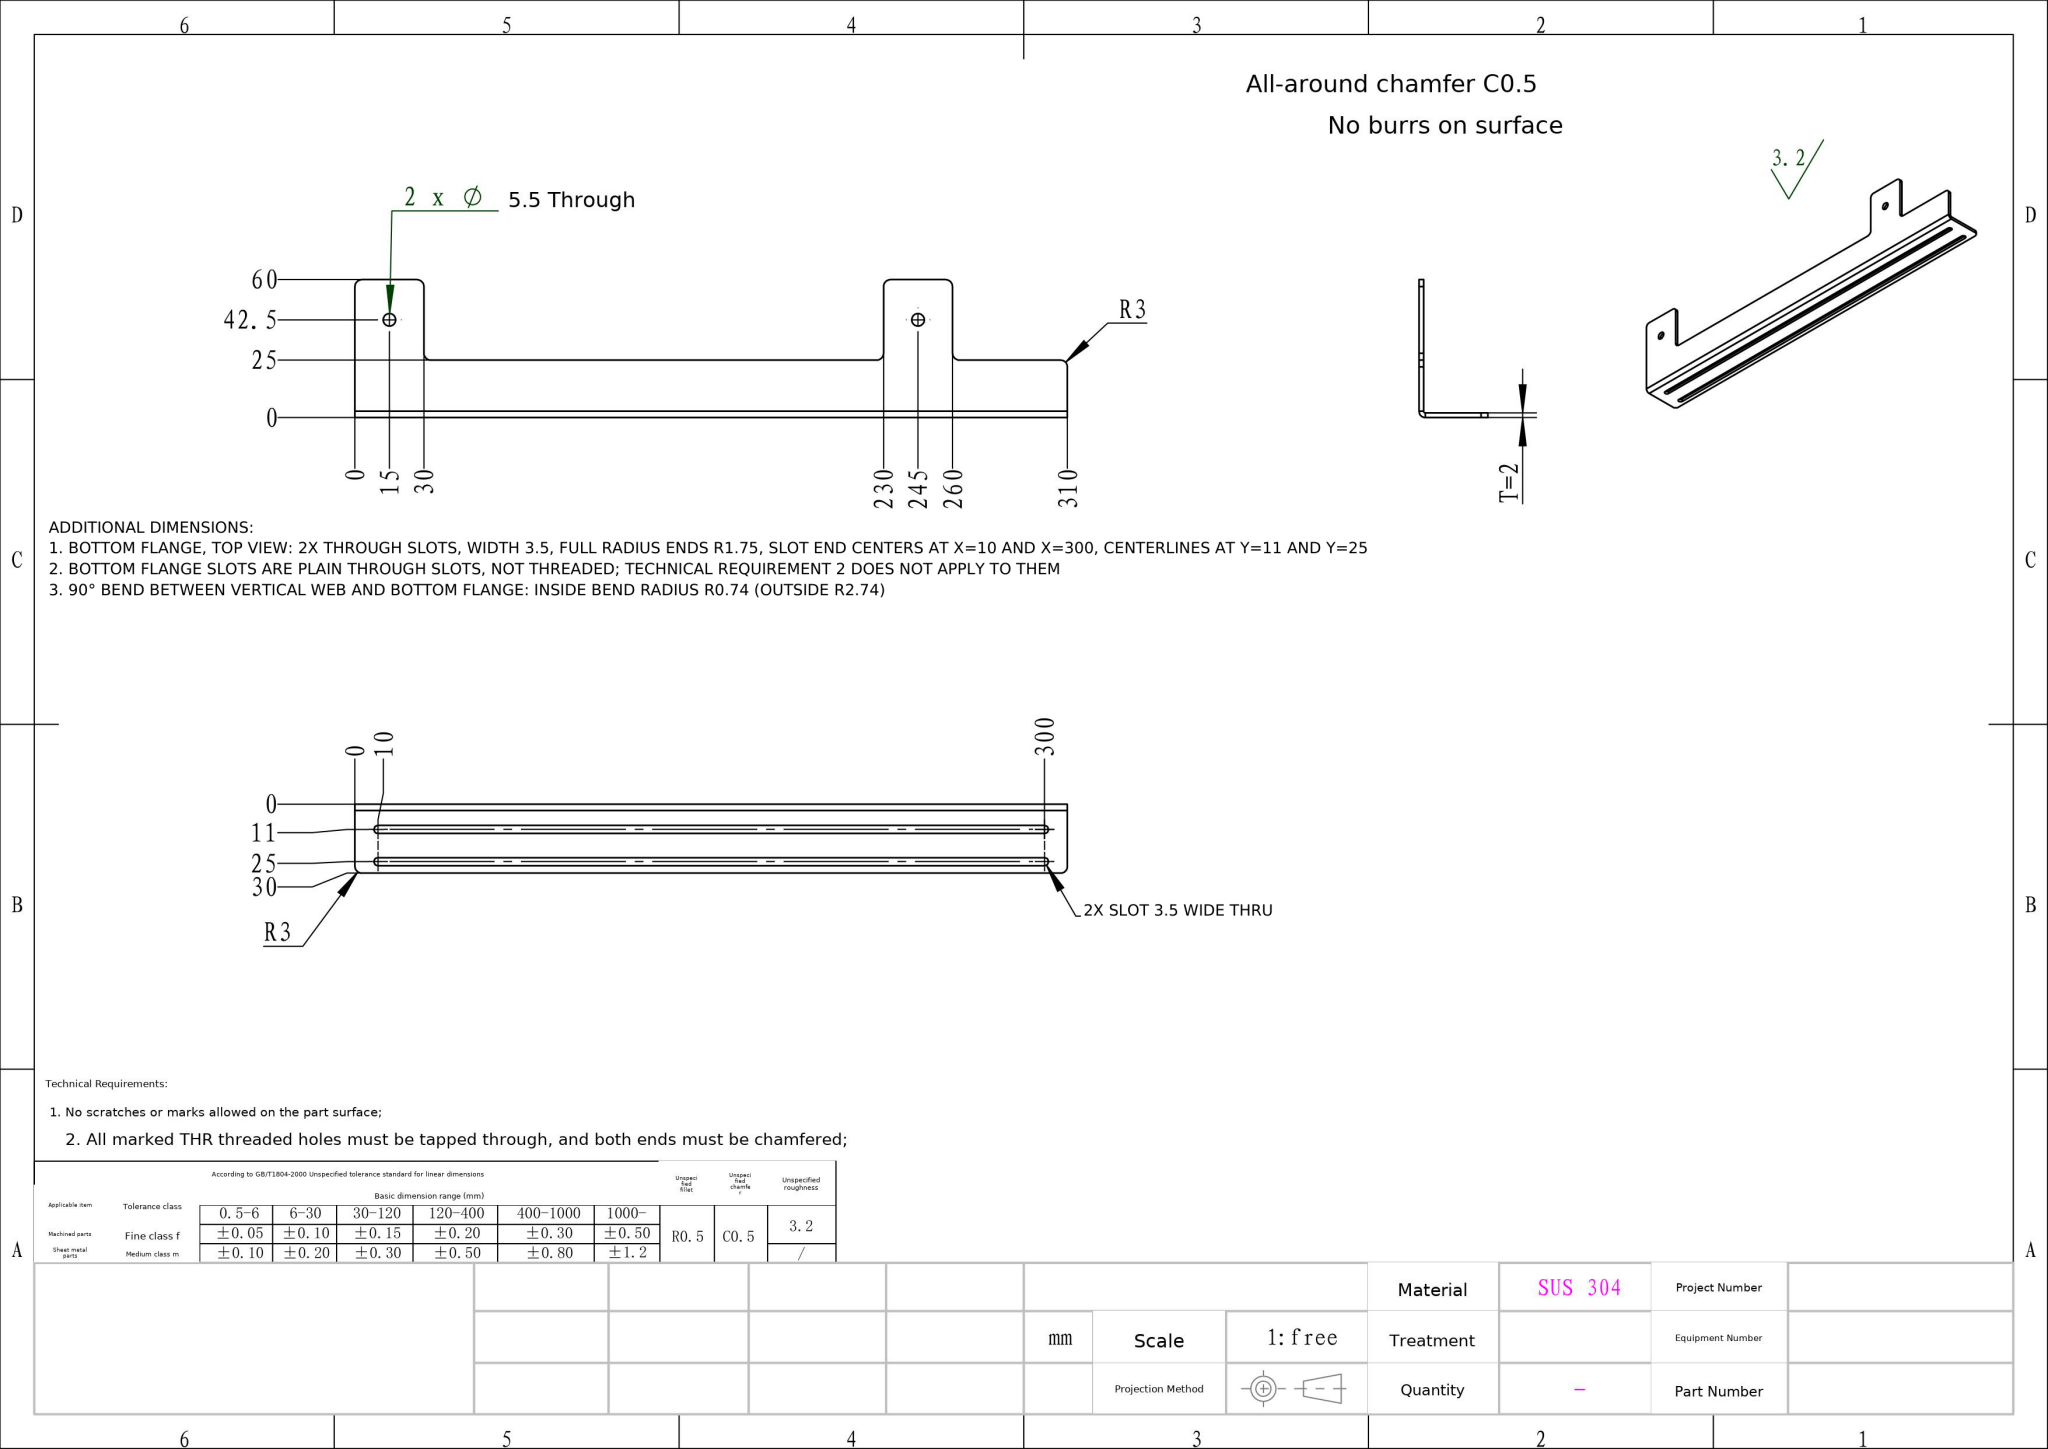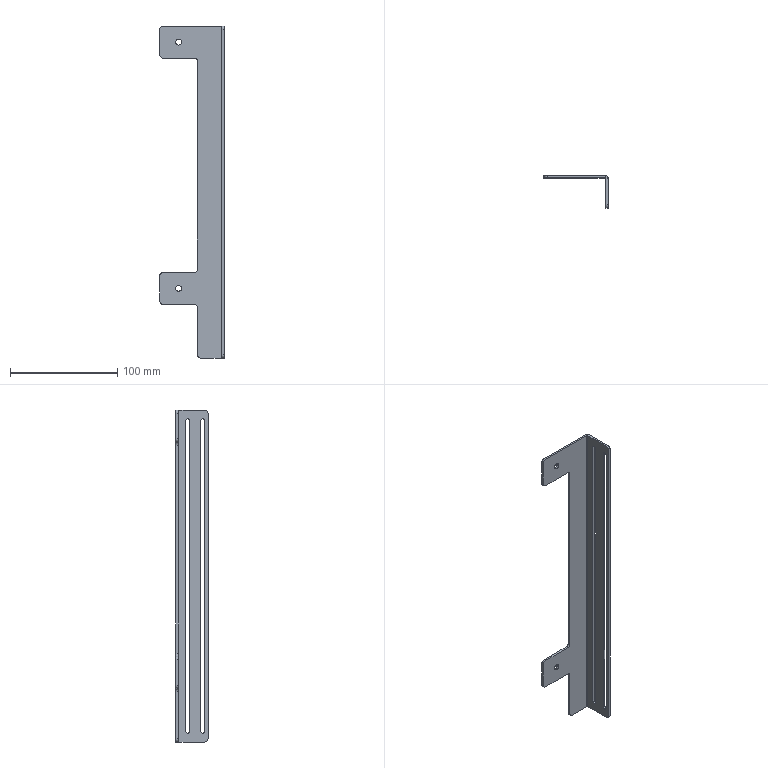Part | NX | mm | 1 solid | 42 faces | box 60 x 30 x 310 mm | volume 32389 mm3 | plane 22 | cylinder 20 | commonest cylinder face diameters 6 x10 5.5 x4 3.5 x4 5.473 x1 1.473 x1